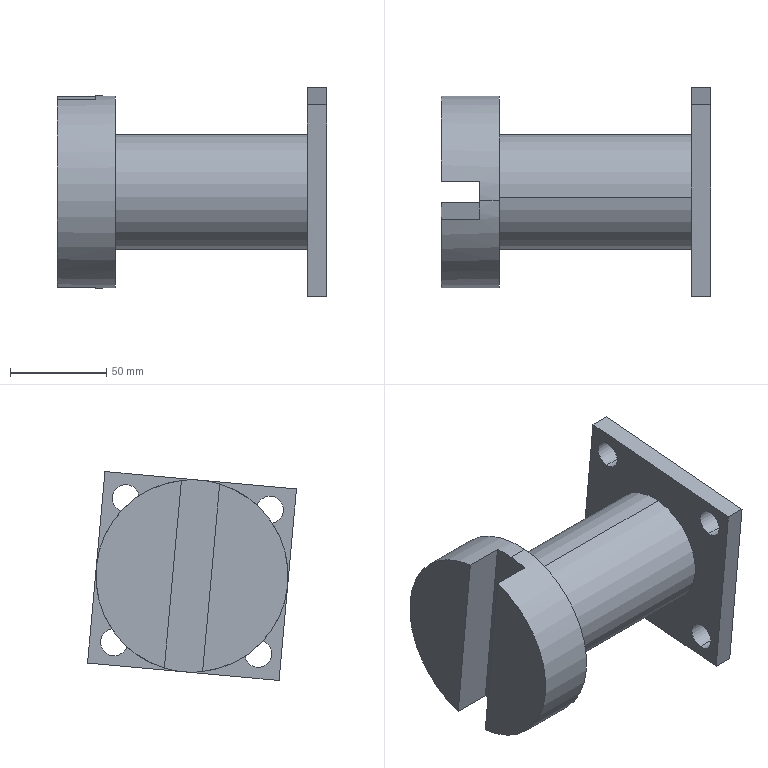Component | SolidWorks | CouplerAssembly-1_LowerCoupler-1 | 1 solid | 27 faces | box 140 x 108.64 x 108.64 mm | volume 570934 mm3 | cylinder 14 | plane 13 | commonest cylinder face diameters 14 x10 60 x2 100 x2
build123d program:
from build123d import *

# Parameters (mm, degrees)
SKETCH1_R           = 50
BOSS_EXTRUDE1_DEPTH = 30
CUT_EXTRUDE1_REACH  = 117.758
SKETCH3_W           = 20
SKETCH3_H           = 20
SKETCH4_R           = 30
BOSS_EXTRUDE2_DEPTH = 100
SKETCH7_W           = 100
SKETCH7_H           = 100
BOSS_EXTRUDE3_DEPTH = 10
SKETCH8_R           = 7
CUT_EXTRUDE4_DEPTH  = 10
CIRPATTERN1_COUNT   = 4
SKETCH9_R           = 7
CUT_EXTRUDE5_DEPTH  = 10


with BuildPart() as part:
    # Sketch1 → Boss-Extrude1 (new body)
    with BuildSketch(Plane.XY):
        Circle(SKETCH1_R)
    extrude(amount=BOSS_EXTRUDE1_DEPTH)

    # Sketch3 → Cut-Extrude1 (cut, up to next)
    with BuildSketch(Plane(origin=(50, 0, 0), x_dir=(0, 0, -1), z_dir=(1, 0, 0)), mode=Mode.PRIVATE) as cut_extrude1_sk1:
        with Locations((-10, 0)):
            Rectangle(SKETCH3_W, SKETCH3_H)
    cut_extrude1_tool1 = extrude(cut_extrude1_sk1.sketch, amount=-CUT_EXTRUDE1_REACH, mode=Mode.PRIVATE) & part.part
    add(cut_extrude1_tool1.solids().sort_by_distance((50, 0, 10))[0], mode=Mode.SUBTRACT)

    # Sketch4 → Boss-Extrude2 (add)
    with BuildSketch(Plane.XY.offset(30)):
        Circle(SKETCH4_R)
    extrude(amount=BOSS_EXTRUDE2_DEPTH)

    # Sketch7 → Boss-Extrude3 (add)
    with BuildSketch(Plane.XY.offset(130)):
        Rectangle(SKETCH7_W, SKETCH7_H)
    extrude(amount=BOSS_EXTRUDE3_DEPTH)

    # Sketch8 → Cut-Extrude4 (cut)
    with BuildSketch(Plane.XY.offset(140)):
        with Locations((38, 37.264)):
            Circle(SKETCH8_R)
    cut_extrude4 = extrude(amount=-CUT_EXTRUDE4_DEPTH, mode=Mode.SUBTRACT)

    # CirPattern1: Cut-Extrude4 ×4 about axis
    cirpattern1_axis = Axis((0, 0, 0), (0, 0, 1))
    for i in range(1, CIRPATTERN1_COUNT):
        add(cut_extrude4.rotate(cirpattern1_axis, i * 360 / CIRPATTERN1_COUNT), mode=Mode.SUBTRACT)

    # Sketch9 → Cut-Extrude5 (cut)
    with BuildSketch(Plane.XY.offset(140)):
        Circle(SKETCH9_R)
    extrude(amount=-CUT_EXTRUDE5_DEPTH, mode=Mode.SUBTRACT)


solid = part.part

# Placed as in the assembly
solid = solid.moved(Location((175.641, 70.663, 0), (5.194, 90, 0)))